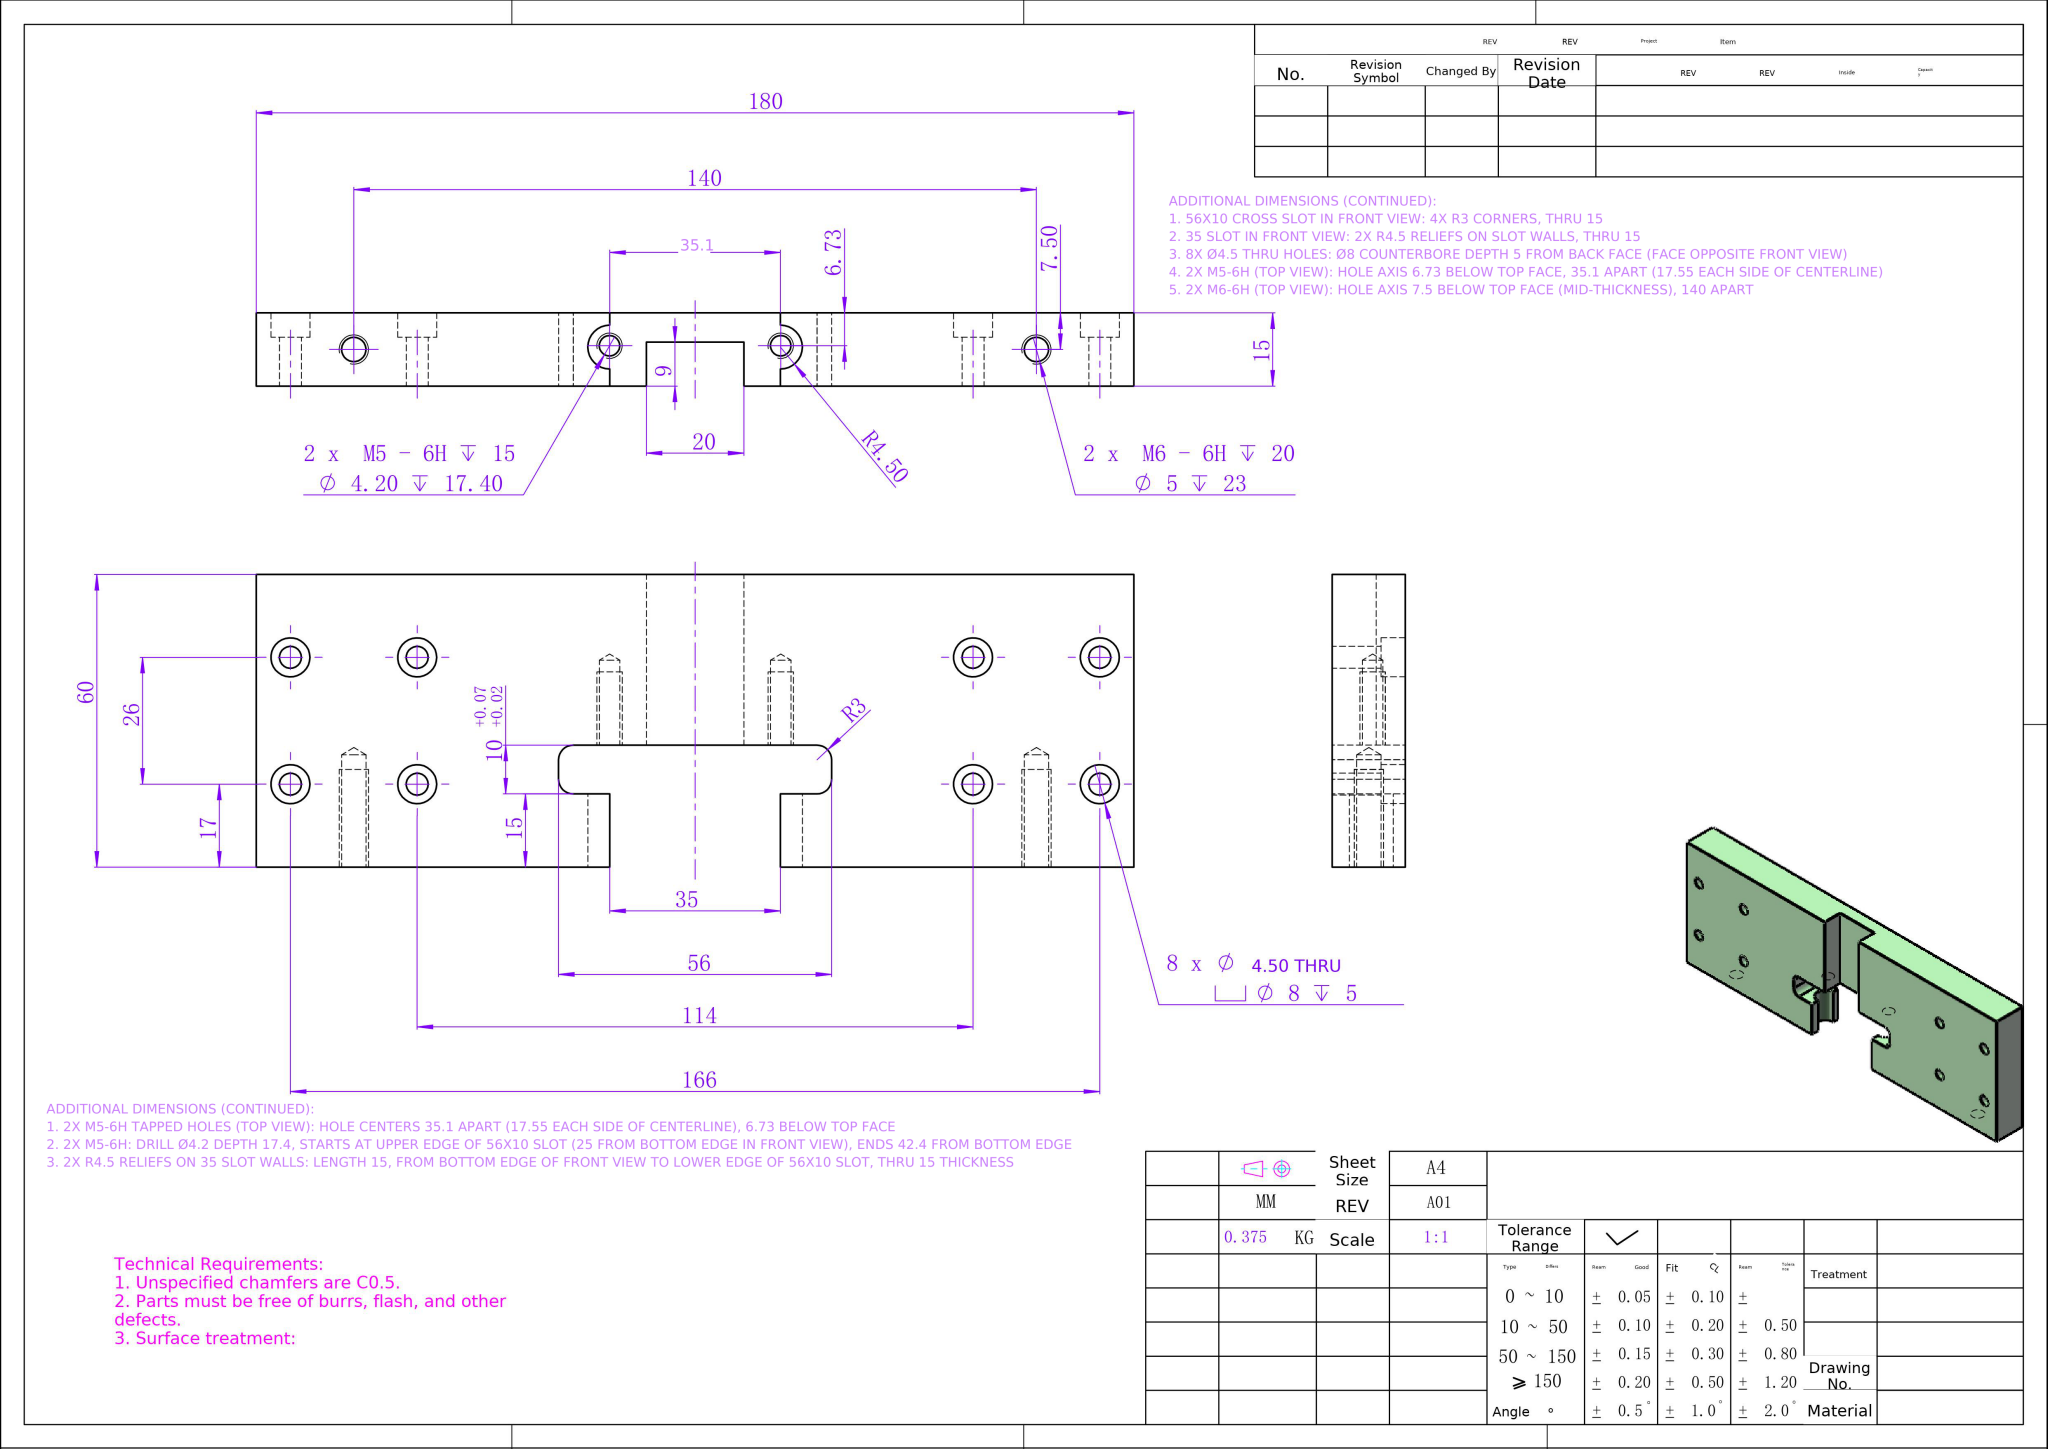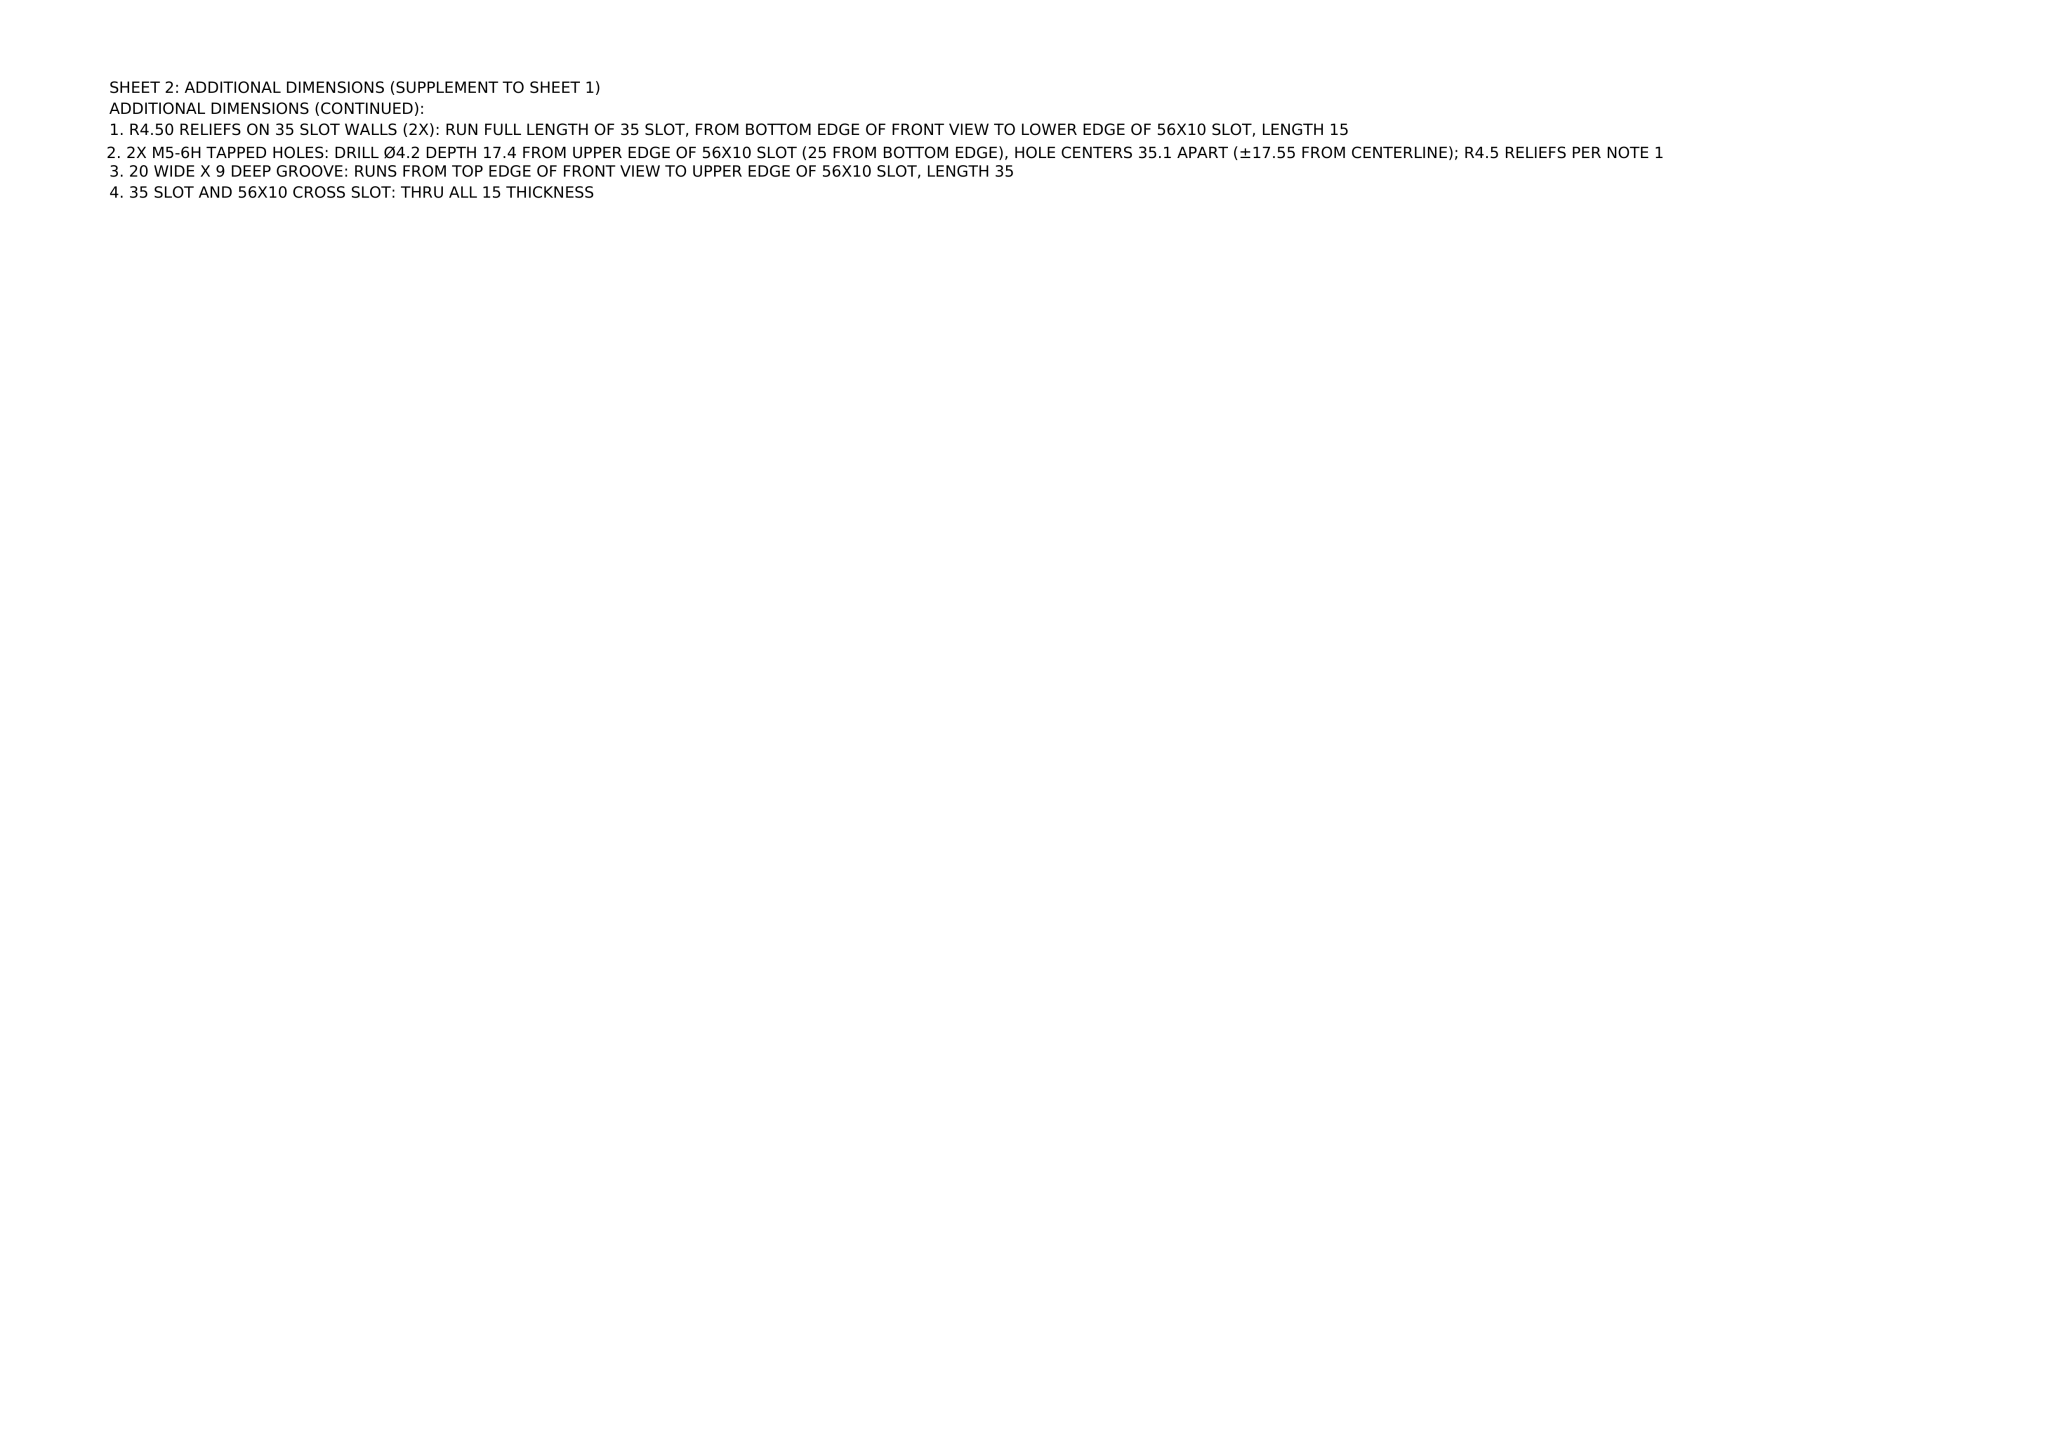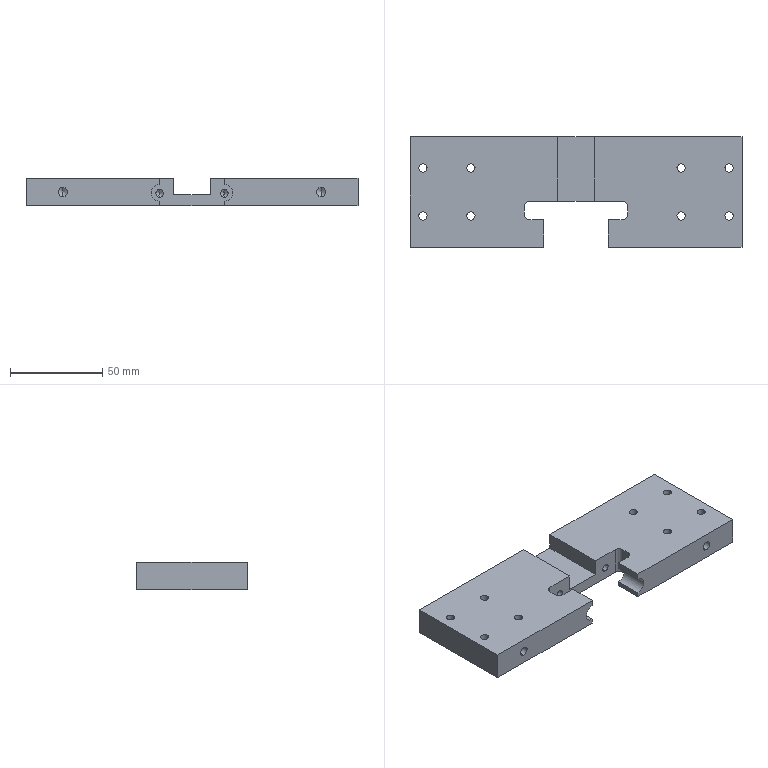Part | NX | mm | 1 solid | 82 faces | box 180 x 60 x 15 mm | volume 133887 mm3 | cylinder 46 | plane 28 | cone 8 | commonest cylinder face diameters 8 x16 4.5 x16 5 x4 4.2 x4 6 x4 9 x2